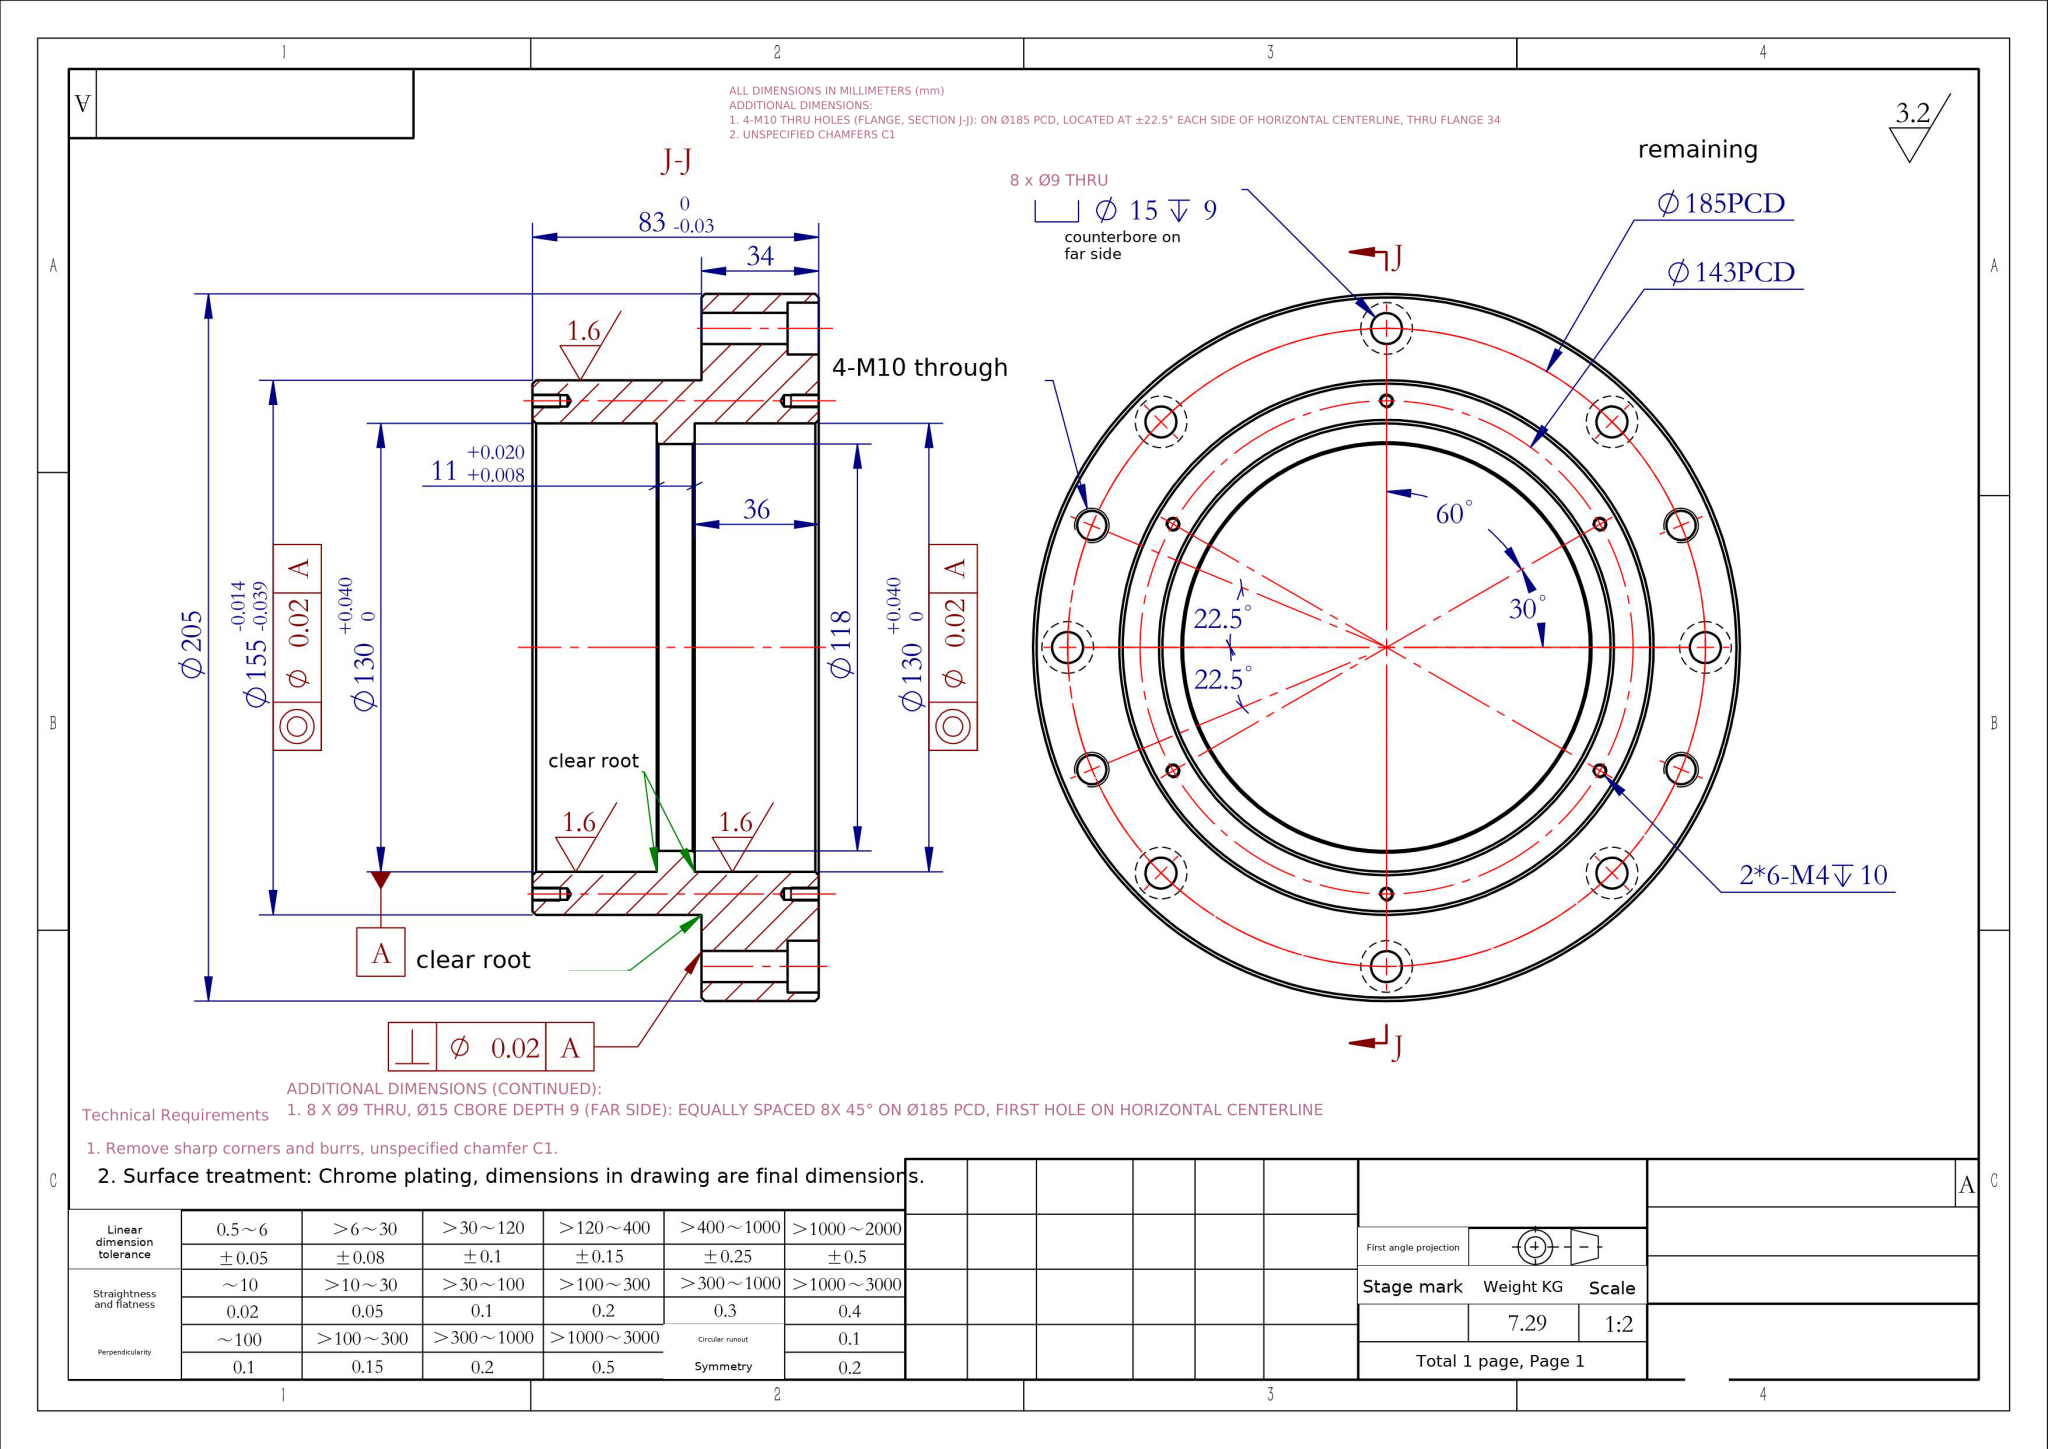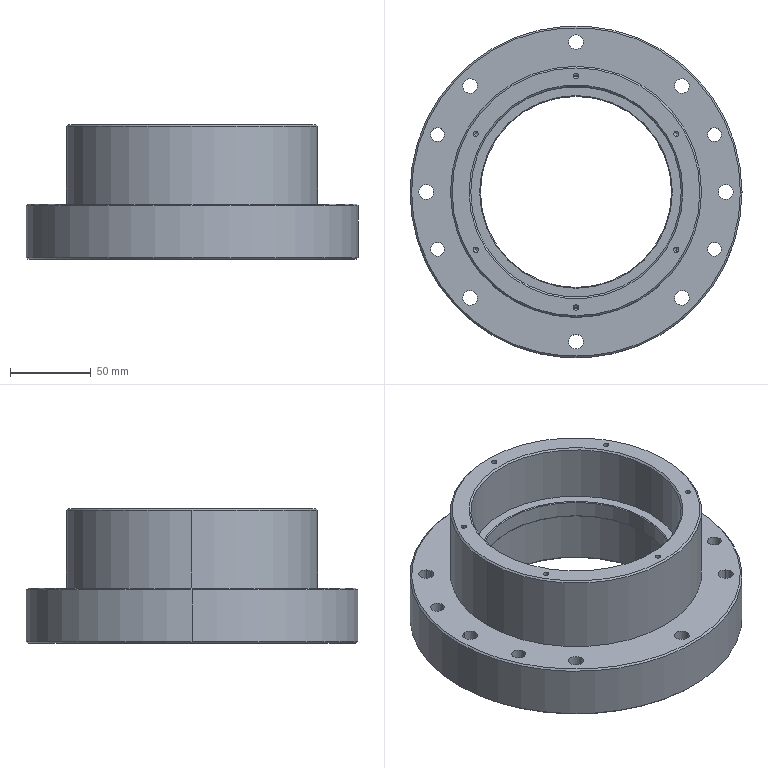Part | NX | mm | 1 solid | 125 faces | box 205 x 205 x 83 mm | volume 935217 mm3 | cylinder 74 | cone 38 | plane 13 | commonest cylinder face diameters 3.3 x24 15 x16 9 x16 8.5 x8 130 x4 155 x2 205 x2 118 x2